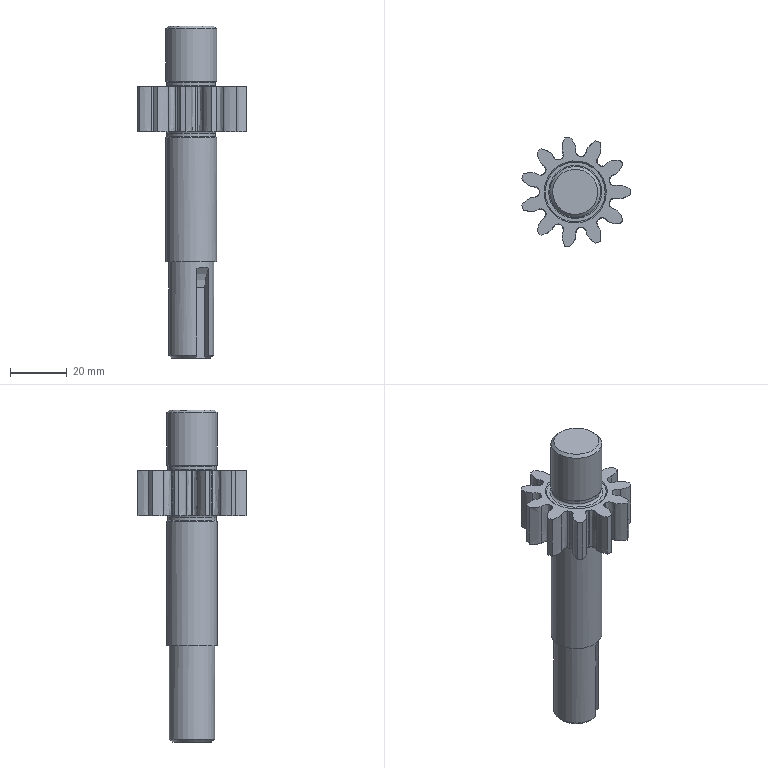Component | NX | 3 | 1 solid | 93 faces | volume 36479 mm3 | other 55 | cylinder 18 | plane 10 | cone 8 | torus 2 | commonest cylinder face diameters 25.5 x11 17.2 x2 18 x2 16 x1 20 x1 1.5 x1